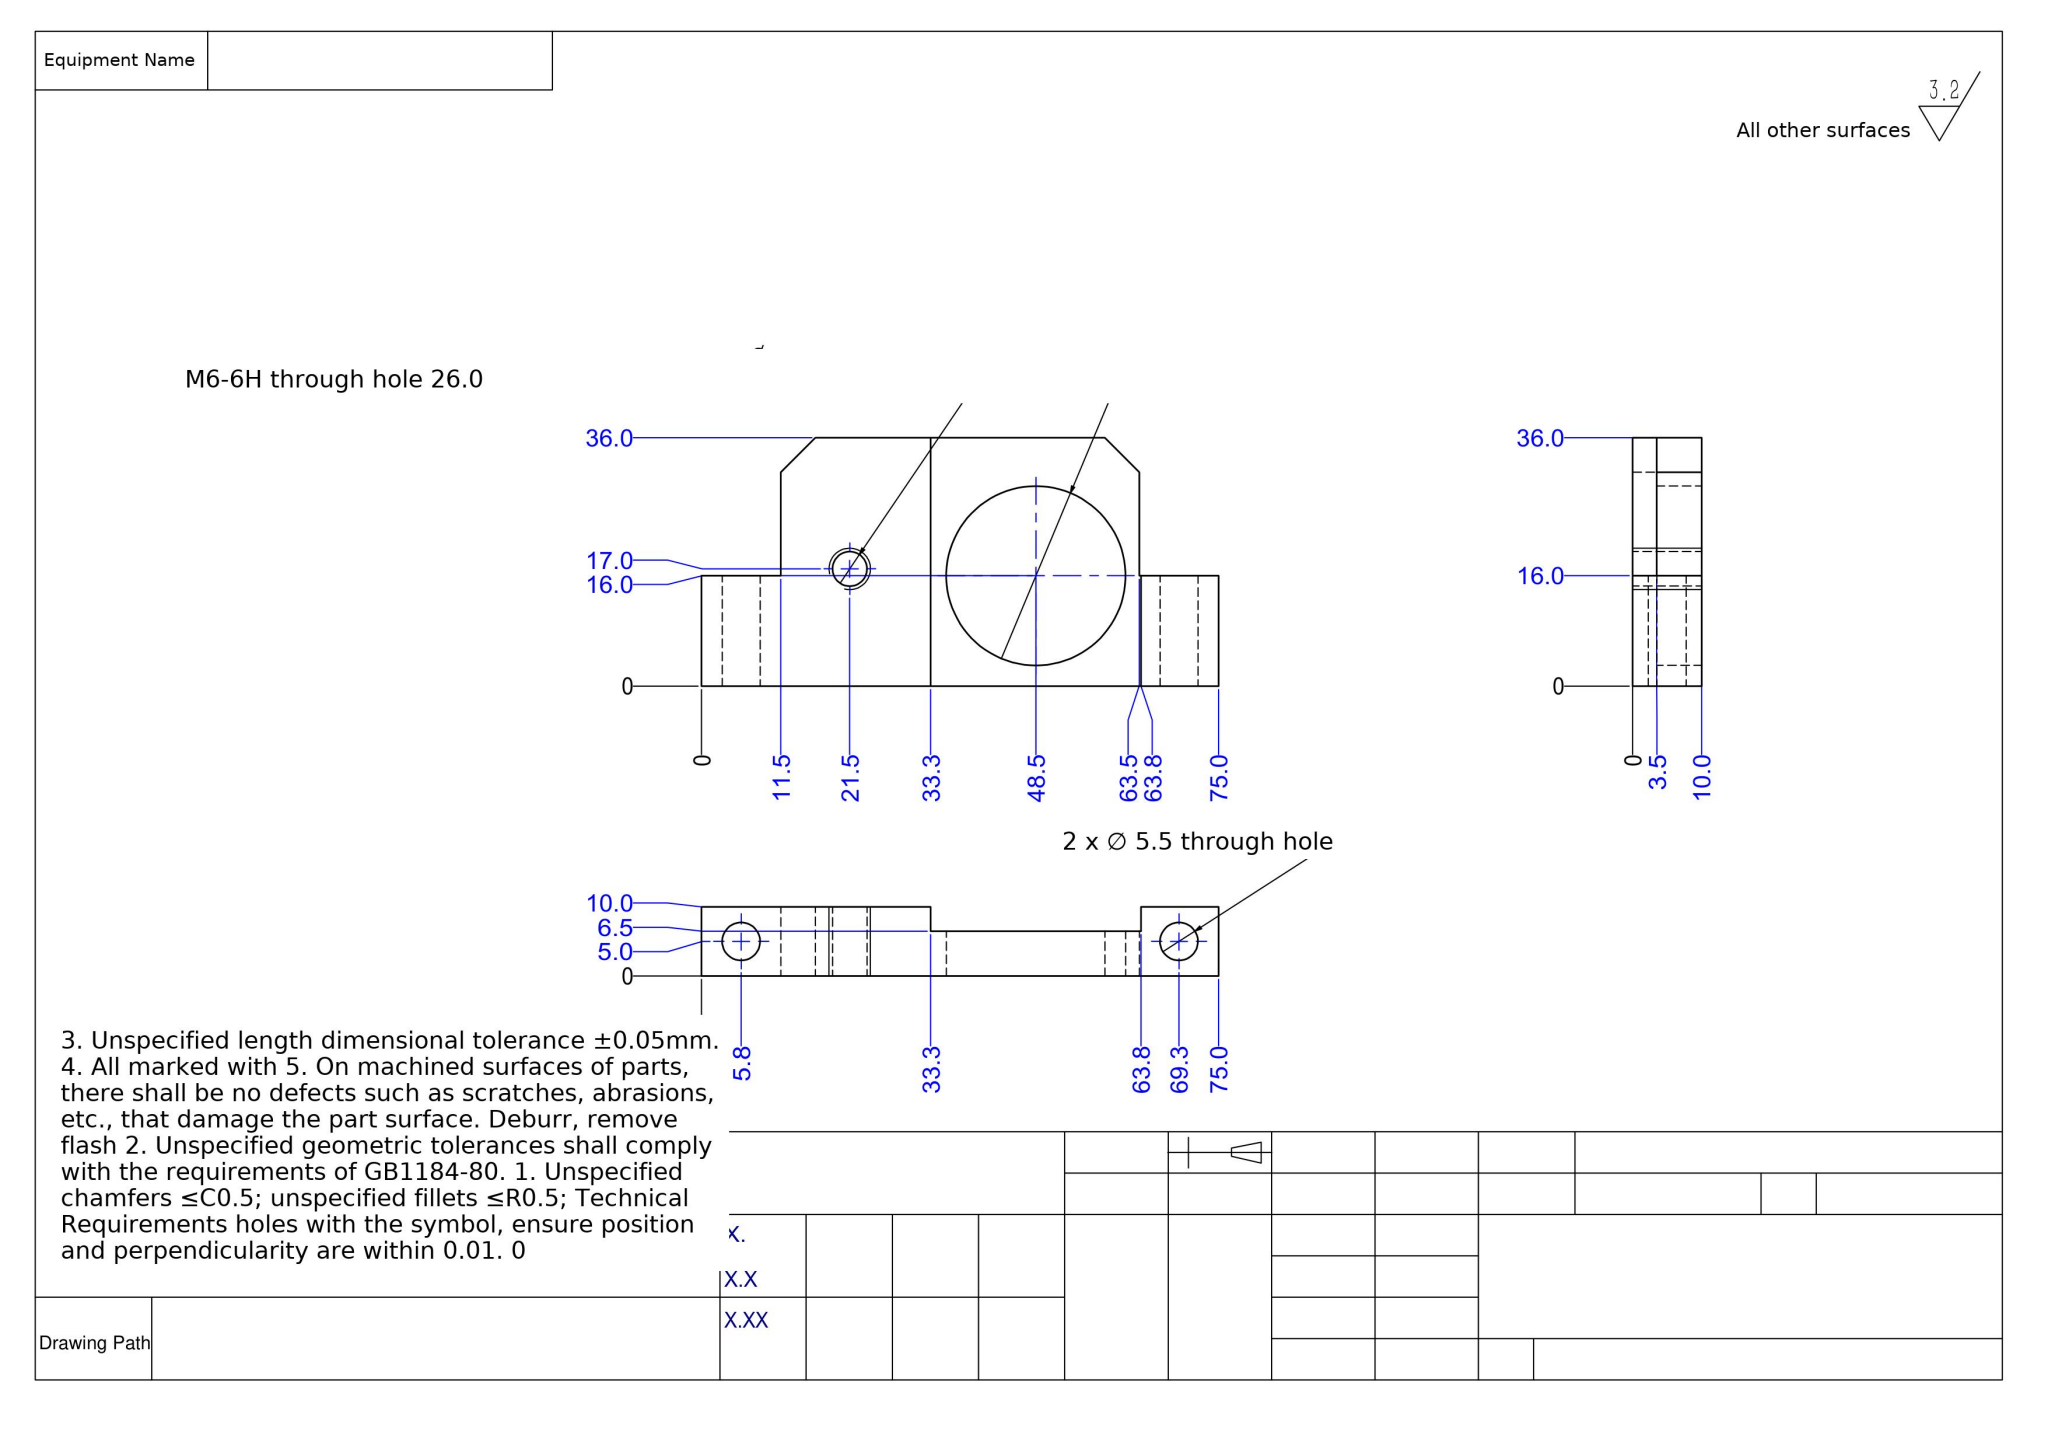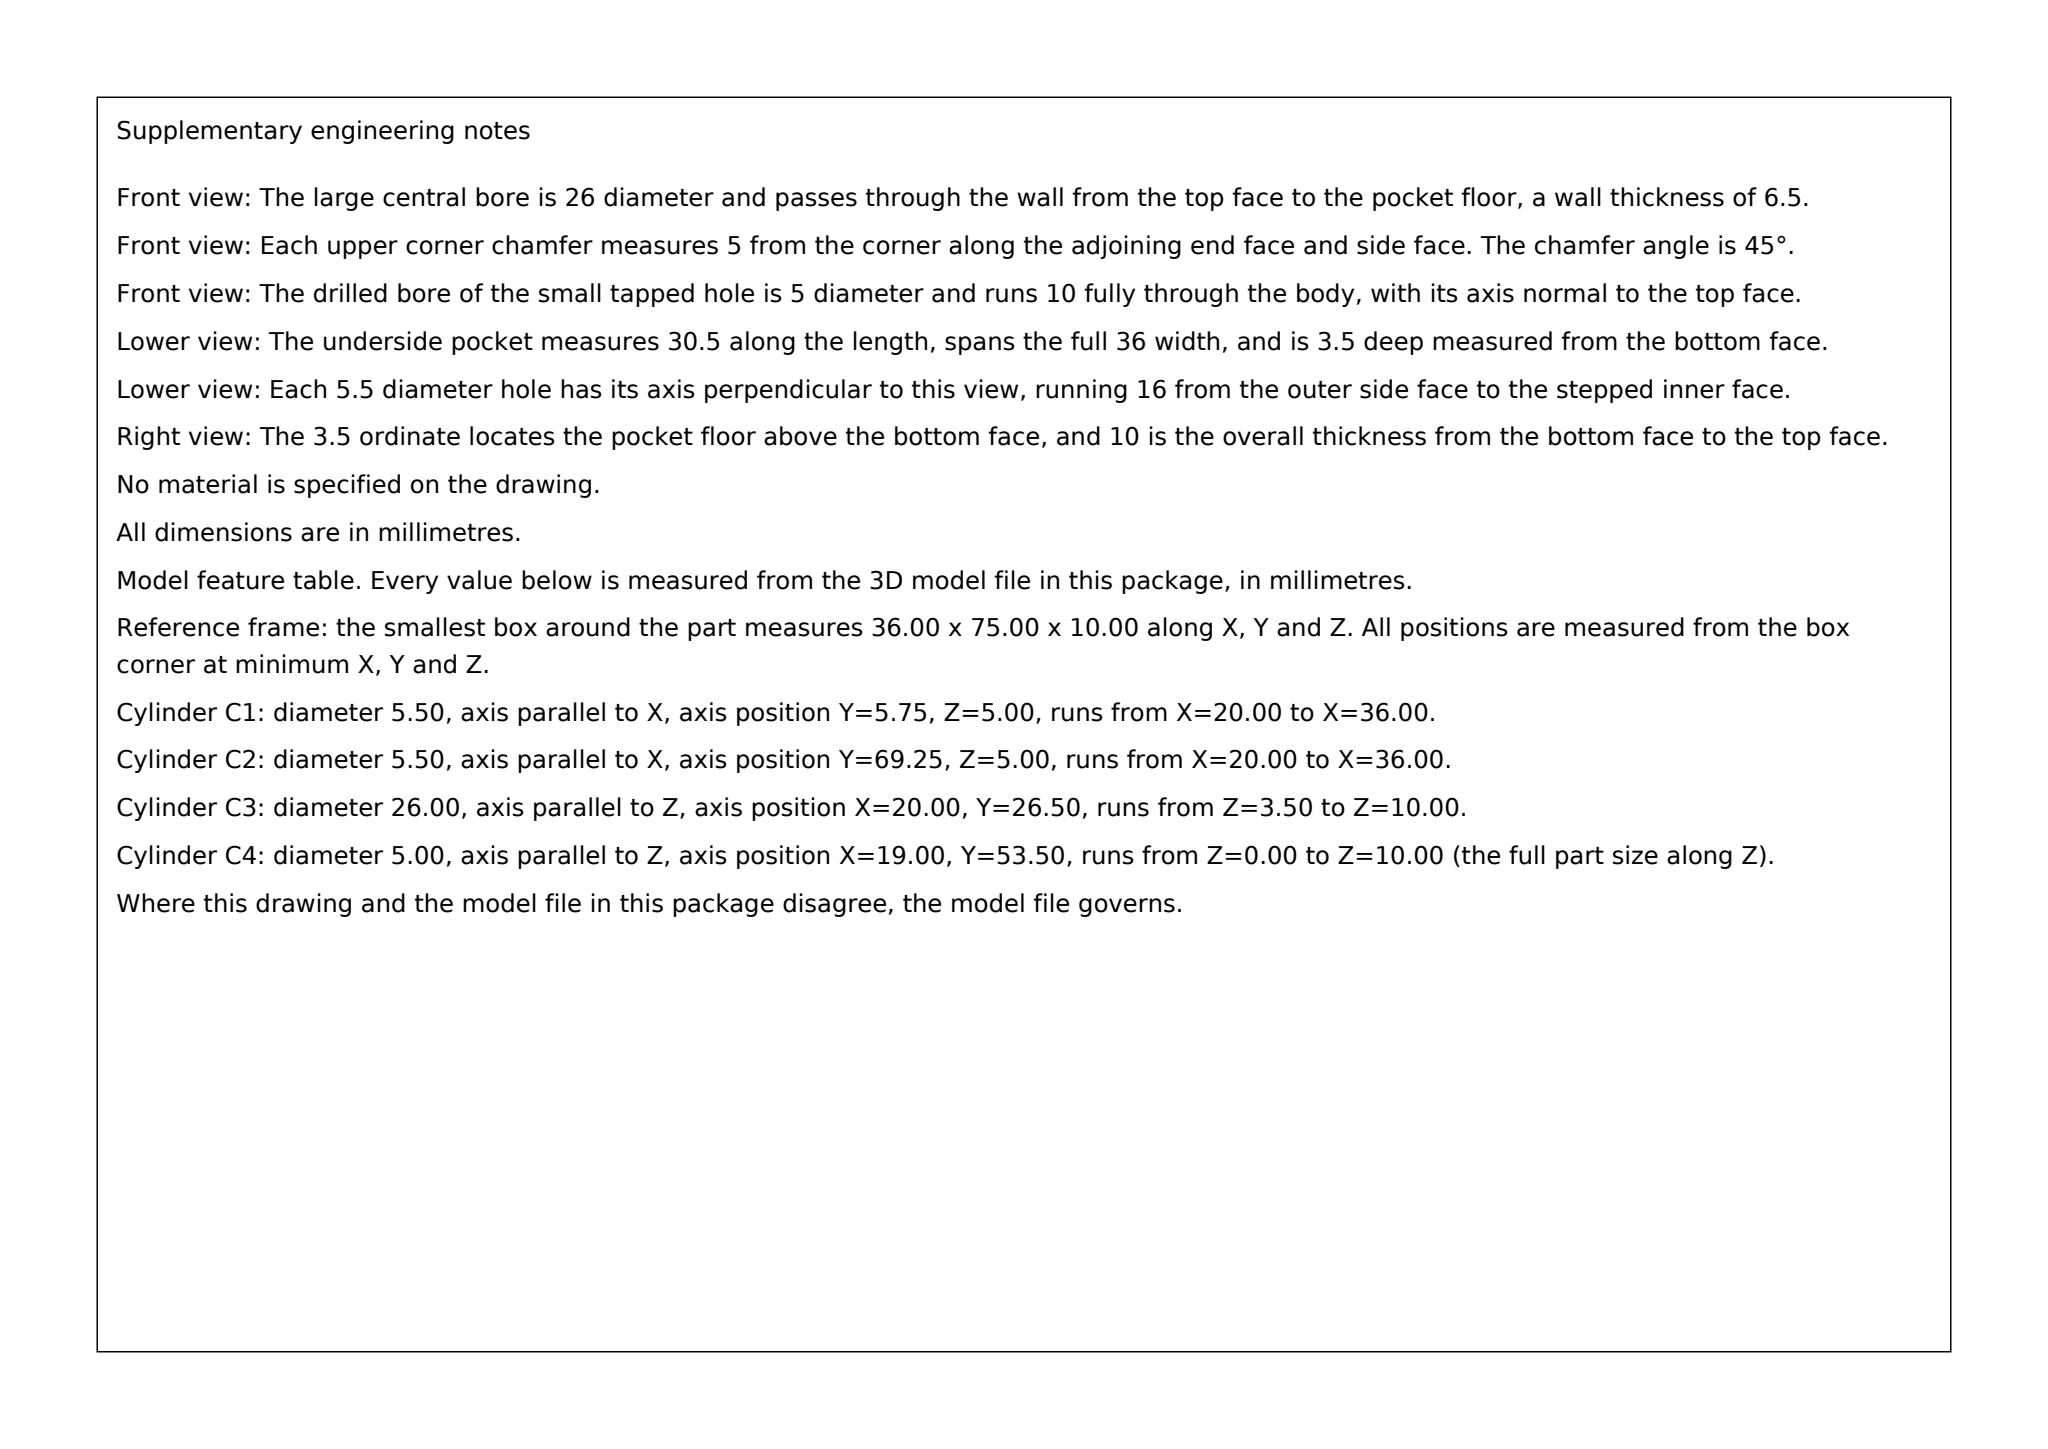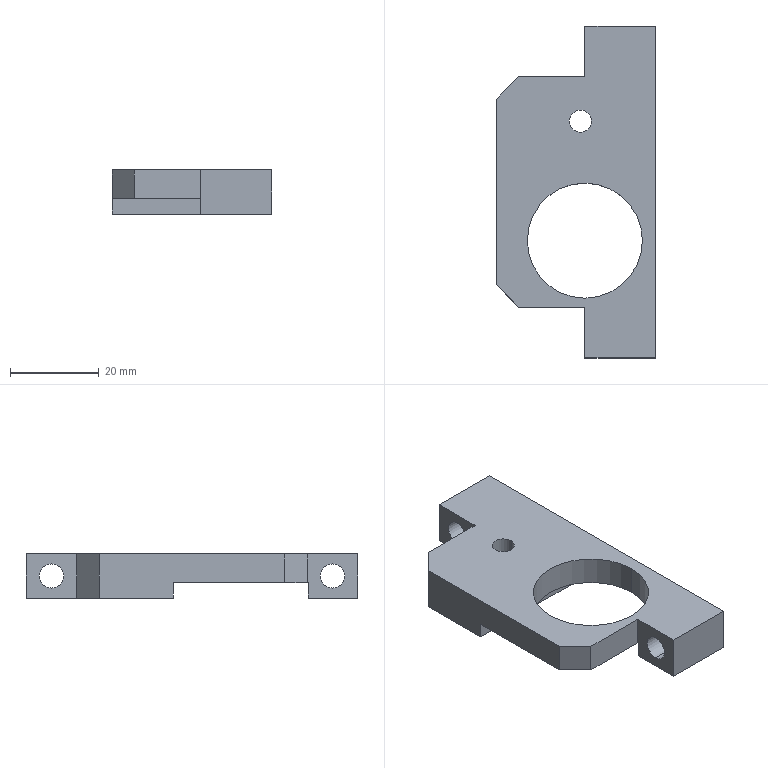Part | SolidWorks | mm | 1 solid | 24 faces | box 36 x 75 x 10 mm | volume 13961 mm3 | plane 16 | cylinder 8 | commonest cylinder face diameters 5.5 x4 5 x2 26 x2
Drawing notes:
FRONT VIEW: 2 X C5 ON TOP CORNERS OF 36.0 FACE (AT 11.5 & 63.5) | from the solid: Top face (x=0 plane, drawing 36.0) spans y 16.5-58.5 between the 11.5 and 63.5 side faces (step y=63.5 / 11.5), i.e. 5 mm x 45 deg cut at each top corner of the 52 wide block.
Ø26 BORE DP 6.5 FROM TOP FACE, CL AT 48.5; FLOOR AT 3.5 | from the solid: cyl dia 26, axis z, pos (20,26.5), len 6.5; z planes 3.5 & 10.0; 75-26.5=48.5
Ø5.0 THRU, CL AT 21.5 & 17.0 (FRONT VIEW) | from the solid: cyl dia 5.0, axis z, pos (19,53.5), len 10.0 = full 10 thk; 75-53.5=21.5, 36-19=17.0
TECH REQ: MARKED HOLES POS & PERP W/IN 0.01; LEN TOL ±0.05 | from the solid: note block text; Ø5.0 THRU holes full 10 thk through part, bbox 36x75x10
build123d program:
from build123d import *

# Parameters (mm, degrees)
SKETCH1_W            = 36
SKETCH1_H            = 75
BOSS_EXTRUDE1_DEPTH  = 10
SKETCH2_W            = 20
SKETCH2_H            = 11.5
CUT_EXTRUDE1_DEPTH   = 43.781
SKETCH3_R            = 13
CUT_EXTRUDE2_DEPTH   = 43.781
M6_TAPPED_HOLE1_D    = 5
CHAMFER1_SIZE        = 5
M5_CLEARANCE_HOLE1_D = 5.5
SKETCH8_W            = 40
SKETCH8_H            = 30.5
CUT_EXTRUDE3_DEPTH   = 3.5


with BuildPart() as part:
    # Sketch1 → Boss-Extrude1 (new body)
    with BuildSketch(Plane.XY):
        Rectangle(SKETCH1_W, SKETCH1_H)
    extrude(amount=BOSS_EXTRUDE1_DEPTH)

    # Sketch2 → Cut-Extrude1 (cut, through all)
    with BuildSketch(Plane.XY.offset(10)):
        with Locations((-8, 31.75)):
            Rectangle(SKETCH2_W, SKETCH2_H)
        with Locations((-8, -31.75)):
            Rectangle(SKETCH2_W, SKETCH2_H)
    extrude(amount=-CUT_EXTRUDE1_DEPTH, mode=Mode.SUBTRACT)

    # Sketch3 → Cut-Extrude2 (cut, through all)
    with BuildSketch(Plane.XY.offset(10)):
        with Locations((2, -11)):
            Circle(SKETCH3_R)
    extrude(amount=-CUT_EXTRUDE2_DEPTH, mode=Mode.SUBTRACT)

    # M6 Tapped Hole1 (through all)
    with Locations(Plane.XY.offset(10)):
        with Locations((1, 16)):
            Hole(M6_TAPPED_HOLE1_D / 2)

    # Chamfer1
    chamfer1_edges = [part.edges().sort_by_distance(p)[0] for p in [
        (-18, 26, 5),
        (-18, -26, 5),
    ]]
    chamfer(chamfer1_edges, length=CHAMFER1_SIZE)

    # M5 Clearance Hole1 (through all)
    with Locations(Plane.ZY.offset(-2)):
        with Locations((5, -31.75), (5, 31.75)):
            Hole(M5_CLEARANCE_HOLE1_D / 2)

    # Sketch8 → Cut-Extrude3 (cut)
    with BuildSketch(Plane(origin=(0, 0, 0), x_dir=(-1, 0, 0), z_dir=(0, 0, -1))):
        with Locations((-2, -11)):
            Rectangle(SKETCH8_W, SKETCH8_H)
    extrude(amount=-CUT_EXTRUDE3_DEPTH, mode=Mode.SUBTRACT)


solid = part.part
STEP:
#1=CARTESIAN_POINT('',(18.,-31.75,2.25));
#2=VERTEX_POINT('',#1);
#3=CARTESIAN_POINT('',(18.,-31.75,7.75));
#4=VERTEX_POINT('',#3);
#5=CARTESIAN_POINT('',(18.,-31.75,5.));
#6=DIRECTION('',(-1.,0.,0.));
#7=DIRECTION('',(0.,0.,1.));
#8=AXIS2_PLACEMENT_3D('',#5,#6,#7);
#9=CIRCLE('',#8,2.75);
#10=EDGE_CURVE('',#2,#4,#9,.T.);
#11=ORIENTED_EDGE('',*,*,#10,.F.);
#12=CARTESIAN_POINT('',(2.,-31.75,2.25));
#13=VERTEX_POINT('',#12);
#14=CARTESIAN_POINT('',(2.,-31.75,2.25));
#15=DIRECTION('',(-1.,0.,0.));
#16=VECTOR('',#15,1000.);
#17=LINE('',#14,#16);
#18=EDGE_CURVE('',#2,#13,#17,.T.);
#19=ORIENTED_EDGE('',*,*,#18,.T.);
#20=CARTESIAN_POINT('',(2.,-31.75,7.75));
#21=VERTEX_POINT('',#20);
#22=CARTESIAN_POINT('',(2.,-31.75,5.));
#23=DIRECTION('',(-1.,0.,0.));
#24=DIRECTION('',(0.,0.,1.));
#25=AXIS2_PLACEMENT_3D('',#22,#23,#24);
#26=CIRCLE('',#25,2.75);
#27=EDGE_CURVE('',#13,#21,#26,.T.);
#28=ORIENTED_EDGE('',*,*,#27,.T.);
#29=CARTESIAN_POINT('',(2.,-31.75,7.75));
#30=DIRECTION('',(-1.,0.,0.));
#31=VECTOR('',#30,1000.);
#32=LINE('',#29,#31);
#33=EDGE_CURVE('',#4,#21,#32,.T.);
#34=ORIENTED_EDGE('',*,*,#33,.F.);
#35=EDGE_LOOP('',(#11,#19,#28,#34));
#36=FACE_OUTER_BOUND('',#35,.T.);
#37=CARTESIAN_POINT('',(2.,-31.75,5.));
#38=DIRECTION('',(-1.,0.,0.));
#39=DIRECTION('',(0.,0.,1.));
#40=AXIS2_PLACEMENT_3D('',#37,#38,#39);
#41=CYLINDRICAL_SURFACE('',#40,2.75);
#42=ADVANCED_FACE('',(#36),#41,.F.);
#43=CARTESIAN_POINT('',(18.,31.75,2.25));
#44=VERTEX_POINT('',#43);
#45=CARTESIAN_POINT('',(18.,31.75,7.75));
#46=VERTEX_POINT('',#45);
#47=CARTESIAN_POINT('',(18.,31.75,5.));
#48=DIRECTION('',(-1.,0.,0.));
#49=DIRECTION('',(0.,0.,1.));
#50=AXIS2_PLACEMENT_3D('',#47,#48,#49);
#51=CIRCLE('',#50,2.75);
#52=EDGE_CURVE('',#44,#46,#51,.T.);
#53=ORIENTED_EDGE('',*,*,#52,.F.);
#54=CARTESIAN_POINT('',(2.,31.75,2.25));
#55=VERTEX_POINT('',#54);
#56=CARTESIAN_POINT('',(2.,31.75,2.25));
#57=DIRECTION('',(-1.,0.,0.));
#58=VECTOR('',#57,1000.);
#59=LINE('',#56,#58);
#60=EDGE_CURVE('',#44,#55,#59,.T.);
#61=ORIENTED_EDGE('',*,*,#60,.T.);
#62=CARTESIAN_POINT('',(2.,31.75,7.75));
#63=VERTEX_POINT('',#62);
#64=CARTESIAN_POINT('',(2.,31.75,5.));
#65=DIRECTION('',(-1.,0.,0.));
#66=DIRECTION('',(0.,0.,1.));
#67=AXIS2_PLACEMENT_3D('',#64,#65,#66);
#68=CIRCLE('',#67,2.75);
#69=EDGE_CURVE('',#55,#63,#68,.T.);
#70=ORIENTED_EDGE('',*,*,#69,.T.);
#71=CARTESIAN_POINT('',(2.,31.75,7.75));
#72=DIRECTION('',(-1.,0.,0.));
#73=VECTOR('',#72,1000.);
#74=LINE('',#71,#73);
#75=EDGE_CURVE('',#46,#63,#74,.T.);
#76=ORIENTED_EDGE('',*,*,#75,.F.);
#77=EDGE_LOOP('',(#53,#61,#70,#76));
#78=FACE_OUTER_BOUND('',#77,.T.);
#79=CARTESIAN_POINT('',(2.,31.75,5.));
#80=DIRECTION('',(-1.,0.,0.));
#81=DIRECTION('',(0.,0.,1.));
#82=AXIS2_PLACEMENT_3D('',#79,#80,#81);
#83=CYLINDRICAL_SURFACE('',#82,2.75);
#84=ADVANCED_FACE('',(#78),#83,.F.);
#85=CARTESIAN_POINT('',(-1.5,16.,0.));
#86=VERTEX_POINT('',#85);
#87=CARTESIAN_POINT('',(3.5,16.,0.));
#88=VERTEX_POINT('',#87);
#89=CARTESIAN_POINT('',(1.,16.,0.));
#90=DIRECTION('',(0.,0.,1.));
#91=DIRECTION('',(1.,0.,0.));
#92=AXIS2_PLACEMENT_3D('',#89,#90,#91);
#93=CIRCLE('',#92,2.5);
#94=EDGE_CURVE('',#86,#88,#93,.T.);
#95=ORIENTED_EDGE('',*,*,#94,.F.);
#96=CARTESIAN_POINT('',(-1.5,16.,10.));
#97=VERTEX_POINT('',#96);
#98=CARTESIAN_POINT('',(-1.5,16.,10.));
#99=DIRECTION('',(0.,0.,1.));
#100=VECTOR('',#99,1000.);
#101=LINE('',#98,#100);
#102=EDGE_CURVE('',#86,#97,#101,.T.);
#103=ORIENTED_EDGE('',*,*,#102,.T.);
#104=CARTESIAN_POINT('',(3.5,16.,10.));
#105=VERTEX_POINT('',#104);
#106=CARTESIAN_POINT('',(1.,16.,10.));
#107=DIRECTION('',(0.,0.,1.));
#108=DIRECTION('',(1.,0.,0.));
#109=AXIS2_PLACEMENT_3D('',#106,#107,#108);
#110=CIRCLE('',#109,2.5);
#111=EDGE_CURVE('',#97,#105,#110,.T.);
#112=ORIENTED_EDGE('',*,*,#111,.T.);
#113=CARTESIAN_POINT('',(3.5,16.,10.));
#114=DIRECTION('',(0.,0.,1.));
#115=VECTOR('',#114,1000.);
#116=LINE('',#113,#115);
#117=EDGE_CURVE('',#88,#105,#116,.T.);
#118=ORIENTED_EDGE('',*,*,#117,.F.);
#119=EDGE_LOOP('',(#95,#103,#112,#118));
#120=FACE_OUTER_BOUND('',#119,.T.);
#121=CARTESIAN_POINT('',(1.,16.,10.));
#122=DIRECTION('',(0.,0.,1.));
#123=DIRECTION('',(1.,0.,0.));
#124=AXIS2_PLACEMENT_3D('',#121,#122,#123);
#125=CYLINDRICAL_SURFACE('',#124,2.5);
#126=ADVANCED_FACE('',(#120),#125,.F.);
#127=CARTESIAN_POINT('',(-11.,-11.,3.5));
#128=VERTEX_POINT('',#127);
#129=CARTESIAN_POINT('',(15.,-11.,3.5));
#130=VERTEX_POINT('',#129);
#131=CARTESIAN_POINT('',(2.,-11.,3.5));
#132=DIRECTION('',(0.,0.,1.));
#133=DIRECTION('',(-1.,0.,0.));
#134=AXIS2_PLACEMENT_3D('',#131,#132,#133);
#135=CIRCLE('',#134,13.);
#136=EDGE_CURVE('',#128,#130,#135,.T.);
#137=ORIENTED_EDGE('',*,*,#136,.F.);
#138=CARTESIAN_POINT('',(-11.,-11.,10.));
#139=VERTEX_POINT('',#138);
#140=CARTESIAN_POINT('',(-11.,-11.,0.));
#141=DIRECTION('',(0.,0.,1.));
#142=VECTOR('',#141,1000.);
#143=LINE('',#140,#142);
#144=EDGE_CURVE('',#128,#139,#143,.T.);
#145=ORIENTED_EDGE('',*,*,#144,.T.);
#146=CARTESIAN_POINT('',(15.,-11.,10.));
#147=VERTEX_POINT('',#146);
#148=CARTESIAN_POINT('',(2.,-11.,10.));
#149=DIRECTION('',(0.,0.,1.));
#150=DIRECTION('',(1.,0.,0.));
#151=AXIS2_PLACEMENT_3D('',#148,#149,#150);
#152=CIRCLE('',#151,13.);
#153=EDGE_CURVE('',#139,#147,#152,.T.);
#154=ORIENTED_EDGE('',*,*,#153,.T.);
#155=CARTESIAN_POINT('',(15.,-11.,0.));
#156=DIRECTION('',(0.,0.,1.));
#157=VECTOR('',#156,1000.);
#158=LINE('',#155,#157);
#159=EDGE_CURVE('',#130,#147,#158,.T.);
#160=ORIENTED_EDGE('',*,*,#159,.F.);
#161=EDGE_LOOP('',(#137,#145,#154,#160));
#162=FACE_OUTER_BOUND('',#161,.T.);
#163=CARTESIAN_POINT('',(2.,-11.,0.));
#164=DIRECTION('',(0.,0.,1.));
#165=DIRECTION('',(1.,0.,0.));
#166=AXIS2_PLACEMENT_3D('',#163,#164,#165);
#167=CYLINDRICAL_SURFACE('',#166,13.);
#168=ADVANCED_FACE('',(#162),#167,.F.);
#169=CARTESIAN_POINT('',(2.,-37.5,0.));
#170=VERTEX_POINT('',#169);
#171=CARTESIAN_POINT('',(2.,-26.25,0.));
#172=VERTEX_POINT('',#171);
#173=CARTESIAN_POINT('',(2.,-37.5,0.));
#174=DIRECTION('',(0.,1.,0.));
#175=VECTOR('',#174,1000.);
#176=LINE('',#173,#175);
#177=EDGE_CURVE('',#170,#172,#176,.T.);
#178=ORIENTED_EDGE('',*,*,#177,.T.);
#179=CARTESIAN_POINT('',(18.,-26.25,0.));
#180=VERTEX_POINT('',#179);
#181=CARTESIAN_POINT('',(22.,-26.25,0.));
#182=DIRECTION('',(-1.,0.,0.));
#183=VECTOR('',#182,1000.);
#184=LINE('',#181,#183);
#185=EDGE_CURVE('',#180,#172,#184,.T.);
#186=ORIENTED_EDGE('',*,*,#185,.F.);
#187=CARTESIAN_POINT('',(18.,-37.5,0.));
#188=VERTEX_POINT('',#187);
#189=CARTESIAN_POINT('',(18.,37.5,0.));
#190=DIRECTION('',(-0.,1.,0.));
#191=VECTOR('',#190,1000.);
#192=LINE('',#189,#191);
#193=EDGE_CURVE('',#188,#180,#192,.T.);
#194=ORIENTED_EDGE('',*,*,#193,.F.);
#195=CARTESIAN_POINT('',(-18.,-37.5,0.));
#196=DIRECTION('',(1.,0.,0.));
#197=VECTOR('',#196,1000.);
#198=LINE('',#195,#197);
#199=EDGE_CURVE('',#170,#188,#198,.T.);
#200=ORIENTED_EDGE('',*,*,#199,.F.);
#201=EDGE_LOOP('',(#178,#186,#194,#200));
#202=FACE_OUTER_BOUND('',#201,.T.);
#203=CARTESIAN_POINT('',(0.,0.,0.));
#204=DIRECTION('',(0.,0.,1.));
#205=DIRECTION('',(1.,0.,0.));
#206=AXIS2_PLACEMENT_3D('',#203,#204,#205);
#207=PLANE('',#206);
#208=ADVANCED_FACE('',(#202),#207,.F.);
#209=CARTESIAN_POINT('',(2.,-26.,3.5));
#210=VERTEX_POINT('',#209);
#211=CARTESIAN_POINT('',(-13.,-26.,3.5));
#212=VERTEX_POINT('',#211);
#213=CARTESIAN_POINT('',(-18.,-26.,3.5));
#214=DIRECTION('',(-1.,-0.,0.));
#215=VECTOR('',#214,1000.);
#216=LINE('',#213,#215);
#217=EDGE_CURVE('',#210,#212,#216,.T.);
#218=ORIENTED_EDGE('',*,*,#217,.F.);
#219=CARTESIAN_POINT('',(2.,-26.,10.));
#220=VERTEX_POINT('',#219);
#221=CARTESIAN_POINT('',(2.,-26.,0.));
#222=DIRECTION('',(0.,0.,1.));
#223=VECTOR('',#222,1000.);
#224=LINE('',#221,#223);
#225=EDGE_CURVE('',#210,#220,#224,.T.);
#226=ORIENTED_EDGE('',*,*,#225,.T.);
#227=CARTESIAN_POINT('',(-13.,-26.,10.));
#228=VERTEX_POINT('',#227);
#229=CARTESIAN_POINT('',(-18.,-26.,10.));
#230=DIRECTION('',(-1.,-0.,0.));
#231=VECTOR('',#230,1000.);
#232=LINE('',#229,#231);
#233=EDGE_CURVE('',#220,#228,#232,.T.);
#234=ORIENTED_EDGE('',*,*,#233,.T.);
#235=CARTESIAN_POINT('',(-13.,-26.,0.));
#236=DIRECTION('',(0.,0.,-1.));
#237=VECTOR('',#236,1000.);
#238=LINE('',#235,#237);
#239=EDGE_CURVE('',#228,#212,#238,.T.);
#240=ORIENTED_EDGE('',*,*,#239,.T.);
#241=EDGE_LOOP('',(#218,#226,#234,#240));
#242=FACE_OUTER_BOUND('',#241,.T.);
#243=CARTESIAN_POINT('',(-18.,-26.,0.));
#244=DIRECTION('',(-0.,1.,0.));
#245=DIRECTION('',(-1.,-0.,0.));
#246=AXIS2_PLACEMENT_3D('',#243,#244,#245);
#247=PLANE('',#246);
#248=ADVANCED_FACE('',(#242),#247,.F.);
#249=ORIENTED_EDGE('',*,*,#144,.F.);
#250=CARTESIAN_POINT('',(2.,-11.,3.5));
#251=DIRECTION('',(0.,0.,1.));
#252=DIRECTION('',(-1.,0.,0.));
#253=AXIS2_PLACEMENT_3D('',#250,#251,#252);
#254=CIRCLE('',#253,13.);
#255=EDGE_CURVE('',#130,#128,#254,.T.);
#256=ORIENTED_EDGE('',*,*,#255,.F.);
#257=ORIENTED_EDGE('',*,*,#159,.T.);
#258=CARTESIAN_POINT('',(2.,-11.,10.));
#259=DIRECTION('',(0.,0.,1.));
#260=DIRECTION('',(1.,0.,0.));
#261=AXIS2_PLACEMENT_3D('',#258,#259,#260);
#262=CIRCLE('',#261,13.);
#263=EDGE_CURVE('',#147,#139,#262,.T.);
#264=ORIENTED_EDGE('',*,*,#263,.T.);
#265=EDGE_LOOP('',(#249,#256,#257,#264));
#266=FACE_OUTER_BOUND('',#265,.T.);
#267=CARTESIAN_POINT('',(2.,-11.,0.));
#268=DIRECTION('',(0.,0.,1.));
#269=DIRECTION('',(1.,0.,0.));
#270=AXIS2_PLACEMENT_3D('',#267,#268,#269);
#271=CYLINDRICAL_SURFACE('',#270,13.);
#272=ADVANCED_FACE('',(#266),#271,.F.);
#273=CARTESIAN_POINT('',(-18.,-21.,3.5));
#274=VERTEX_POINT('',#273);
#275=CARTESIAN_POINT('',(-18.,-21.,10.));
#276=VERTEX_POINT('',#275);
#277=CARTESIAN_POINT('',(-18.,-21.,10.));
#278=DIRECTION('',(0.,0.,1.));
#279=VECTOR('',#278,1000.);
#280=LINE('',#277,#279);
#281=EDGE_CURVE('',#274,#276,#280,.T.);
#282=ORIENTED_EDGE('',*,*,#281,.F.);
#283=CARTESIAN_POINT('',(-18.,-21.,3.5));
#284=DIRECTION('',(0.7071,-0.7071,0.));
#285=VECTOR('',#284,1000.);
#286=LINE('',#283,#285);
#287=EDGE_CURVE('',#274,#212,#286,.T.);
#288=ORIENTED_EDGE('',*,*,#287,.T.);
#289=ORIENTED_EDGE('',*,*,#239,.F.);
#290=CARTESIAN_POINT('',(-19.5,-19.5,10.));
#291=DIRECTION('',(0.7071,-0.7071,0.));
#292=VECTOR('',#291,1000.);
#293=LINE('',#290,#292);
#294=EDGE_CURVE('',#276,#228,#293,.T.);
#295=ORIENTED_EDGE('',*,*,#294,.F.);
#296=EDGE_LOOP('',(#282,#288,#289,#295));
#297=FACE_OUTER_BOUND('',#296,.T.);
#298=CARTESIAN_POINT('',(-18.,-21.,10.));
#299=DIRECTION('',(0.7071,0.7071,0.));
#300=DIRECTION('',(0.,0.,1.));
#301=AXIS2_PLACEMENT_3D('',#298,#299,#300);
#302=PLANE('',#301);
#303=ADVANCED_FACE('',(#297),#302,.F.);
#304=ORIENTED_EDGE('',*,*,#193,.T.);
#305=CARTESIAN_POINT('',(18.,-26.25,3.5));
#306=VERTEX_POINT('',#305);
#307=CARTESIAN_POINT('',(18.,-26.25,10.));
#308=DIRECTION('',(0.,0.,1.));
#309=VECTOR('',#308,1000.);
#310=LINE('',#307,#309);
#311=EDGE_CURVE('',#180,#306,#310,.T.);
#312=ORIENTED_EDGE('',*,*,#311,.T.);
#313=CARTESIAN_POINT('',(18.,4.25,3.5));
#314=VERTEX_POINT('',#313);
#315=CARTESIAN_POINT('',(18.,37.5,3.5));
#316=DIRECTION('',(0.,-1.,0.));
#317=VECTOR('',#316,1000.);
#318=LINE('',#315,#317);
#319=EDGE_CURVE('',#314,#306,#318,.T.);
#320=ORIENTED_EDGE('',*,*,#319,.F.);
#321=CARTESIAN_POINT('',(18.,4.25,0.));
#322=VERTEX_POINT('',#321);
#323=CARTESIAN_POINT('',(18.,4.25,10.));
#324=DIRECTION('',(0.,0.,-1.));
#325=VECTOR('',#324,1000.);
#326=LINE('',#323,#325);
#327=EDGE_CURVE('',#314,#322,#326,.T.);
#328=ORIENTED_EDGE('',*,*,#327,.T.);
#329=CARTESIAN_POINT('',(18.,37.5,0.));
#330=VERTEX_POINT('',#329);
#331=CARTESIAN_POINT('',(18.,37.5,0.));
#332=DIRECTION('',(-0.,1.,0.));
#333=VECTOR('',#332,1000.);
#334=LINE('',#331,#333);
#335=EDGE_CURVE('',#322,#330,#334,.T.);
#336=ORIENTED_EDGE('',*,*,#335,.T.);
#337=CARTESIAN_POINT('',(18.,37.5,10.));
#338=VERTEX_POINT('',#337);
#339=CARTESIAN_POINT('',(18.,37.5,10.));
#340=DIRECTION('',(0.,0.,-1.));
#341=VECTOR('',#340,1000.);
#342=LINE('',#339,#341);
#343=EDGE_CURVE('',#338,#330,#342,.T.);
#344=ORIENTED_EDGE('',*,*,#343,.F.);
#345=CARTESIAN_POINT('',(18.,-37.5,10.));
#346=VERTEX_POINT('',#345);
#347=CARTESIAN_POINT('',(18.,37.5,10.));
#348=DIRECTION('',(-0.,1.,0.));
#349=VECTOR('',#348,1000.);
#350=LINE('',#347,#349);
#351=EDGE_CURVE('',#346,#338,#350,.T.);
#352=ORIENTED_EDGE('',*,*,#351,.F.);
#353=CARTESIAN_POINT('',(18.,-37.5,10.));
#354=DIRECTION('',(0.,0.,-1.));
#355=VECTOR('',#354,1000.);
#356=LINE('',#353,#355);
#357=EDGE_CURVE('',#346,#188,#356,.T.);
#358=ORIENTED_EDGE('',*,*,#357,.T.);
#359=EDGE_LOOP('',(#304,#312,#320,#328,#336,#344,#352,#358));
#360=FACE_OUTER_BOUND('',#359,.T.);
#361=CARTESIAN_POINT('',(18.,-31.75,5.));
#362=DIRECTION('',(-1.,0.,0.));
#363=DIRECTION('',(0.,0.,1.));
#364=AXIS2_PLACEMENT_3D('',#361,#362,#363);
#365=CIRCLE('',#364,2.75);
#366=EDGE_CURVE('',#4,#2,#365,.T.);
#367=ORIENTED_EDGE('',*,*,#366,.T.);
#368=ORIENTED_EDGE('',*,*,#10,.T.);
#369=EDGE_LOOP('',(#367,#368));
#370=FACE_BOUND('',#369,.T.);
#371=CARTESIAN_POINT('',(18.,31.75,5.));
#372=DIRECTION('',(-1.,0.,0.));
#373=DIRECTION('',(0.,0.,1.));
#374=AXIS2_PLACEMENT_3D('',#371,#372,#373);
#375=CIRCLE('',#374,2.75);
#376=EDGE_CURVE('',#46,#44,#375,.T.);
#377=ORIENTED_EDGE('',*,*,#376,.T.);
#378=ORIENTED_EDGE('',*,*,#52,.T.);
#379=EDGE_LOOP('',(#377,#378));
#380=FACE_BOUND('',#379,.T.);
#381=CARTESIAN_POINT('',(18.,37.5,10.));
#382=DIRECTION('',(-1.,-0.,0.));
#383=DIRECTION('',(0.,-1.,0.));
#384=AXIS2_PLACEMENT_3D('',#381,#382,#383);
#385=PLANE('',#384);
#386=ADVANCED_FACE('',(#360,#370,#380),#385,.F.);
#387=CARTESIAN_POINT('',(2.,37.5,0.));
#388=VERTEX_POINT('',#387);
#389=CARTESIAN_POINT('',(-18.,37.5,0.));
#390=DIRECTION('',(-1.,0.,0.));
#391=VECTOR('',#390,1000.);
#392=LINE('',#389,#391);
#393=EDGE_CURVE('',#330,#388,#392,.T.);
#394=ORIENTED_EDGE('',*,*,#393,.T.);
#395=CARTESIAN_POINT('',(2.,37.5,10.));
#396=VERTEX_POINT('',#395);
#397=CARTESIAN_POINT('',(2.,37.5,0.));
#398=DIRECTION('',(0.,0.,1.));
#399=VECTOR('',#398,1000.);
#400=LINE('',#397,#399);
#401=EDGE_CURVE('',#388,#396,#400,.T.);
#402=ORIENTED_EDGE('',*,*,#401,.T.);
#403=CARTESIAN_POINT('',(-18.,37.5,10.));
#404=DIRECTION('',(-1.,0.,0.));
#405=VECTOR('',#404,1000.);
#406=LINE('',#403,#405);
#407=EDGE_CURVE('',#338,#396,#406,.T.);
#408=ORIENTED_EDGE('',*,*,#407,.F.);
#409=ORIENTED_EDGE('',*,*,#343,.T.);
#410=EDGE_LOOP('',(#394,#402,#408,#409));
#411=FACE_OUTER_BOUND('',#410,.T.);
#412=CARTESIAN_POINT('',(-18.,37.5,10.));
#413=DIRECTION('',(0.,-1.,0.));
#414=DIRECTION('',(0.,0.,-1.));
#415=AXIS2_PLACEMENT_3D('',#412,#413,#414);
#416=PLANE('',#415);
#417=ADVANCED_FACE('',(#411),#416,.F.);
#418=CARTESIAN_POINT('',(-18.,21.,0.));
#419=VERTEX_POINT('',#418);
#420=CARTESIAN_POINT('',(-18.,4.25,0.));
#421=VERTEX_POINT('',#420);
#422=CARTESIAN_POINT('',(-18.,37.5,0.));
#423=DIRECTION('',(0.,-1.,0.));
#424=VECTOR('',#423,1000.);
#425=LINE('',#422,#424);
#426=EDGE_CURVE('',#419,#421,#425,.T.);
#427=ORIENTED_EDGE('',*,*,#426,.T.);
#428=CARTESIAN_POINT('',(-18.,4.25,3.5));
#429=VERTEX_POINT('',#428);
#430=CARTESIAN_POINT('',(-18.,4.25,3.5));
#431=DIRECTION('',(0.,0.,-1.));
#432=VECTOR('',#431,1000.);
#433=LINE('',#430,#432);
#434=EDGE_CURVE('',#429,#421,#433,.T.);
#435=ORIENTED_EDGE('',*,*,#434,.F.);
#436=CARTESIAN_POINT('',(-18.,4.25,3.5));
#437=DIRECTION('',(0.,1.,0.));
#438=VECTOR('',#437,1000.);
#439=LINE('',#436,#438);
#440=EDGE_CURVE('',#274,#429,#439,.T.);
#441=ORIENTED_EDGE('',*,*,#440,.F.);
#442=ORIENTED_EDGE('',*,*,#281,.T.);
#443=CARTESIAN_POINT('',(-18.,21.,10.));
#444=VERTEX_POINT('',#443);
#445=CARTESIAN_POINT('',(-18.,37.5,10.));
#446=DIRECTION('',(0.,-1.,0.));
#447=VECTOR('',#446,1000.);
#448=LINE('',#445,#447);
#449=EDGE_CURVE('',#444,#276,#448,.T.);
#450=ORIENTED_EDGE('',*,*,#449,.F.);
#451=CARTESIAN_POINT('',(-18.,21.,10.));
#452=DIRECTION('',(0.,0.,-1.));
#453=VECTOR('',#452,1000.);
#454=LINE('',#451,#453);
#455=EDGE_CURVE('',#444,#419,#454,.T.);
#456=ORIENTED_EDGE('',*,*,#455,.T.);
#457=EDGE_LOOP('',(#427,#435,#441,#442,#450,#456));
#458=FACE_OUTER_BOUND('',#457,.T.);
#459=CARTESIAN_POINT('',(-18.,37.5,10.));
#460=DIRECTION('',(1.,0.,0.));
#461=DIRECTION('',(-0.,1.,0.));
#462=AXIS2_PLACEMENT_3D('',#459,#460,#461);
#463=PLANE('',#462);
#464=ADVANCED_FACE('',(#458),#463,.F.);
#465=CARTESIAN_POINT('',(2.,-37.5,10.));
#466=VERTEX_POINT('',#465);
#467=CARTESIAN_POINT('',(-18.,-37.5,10.));
#468=DIRECTION('',(1.,0.,0.));
#469=VECTOR('',#468,1000.);
#470=LINE('',#467,#469);
#471=EDGE_CURVE('',#466,#346,#470,.T.);
#472=ORIENTED_EDGE('',*,*,#471,.F.);
#473=CARTESIAN_POINT('',(2.,-37.5,0.));
#474=DIRECTION('',(0.,0.,1.));
#475=VECTOR('',#474,1000.);
#476=LINE('',#473,#475);
#477=EDGE_CURVE('',#170,#466,#476,.T.);
#478=ORIENTED_EDGE('',*,*,#477,.F.);
#479=ORIENTED_EDGE('',*,*,#199,.T.);
#480=ORIENTED_EDGE('',*,*,#357,.F.);
#481=EDGE_LOOP('',(#472,#478,#479,#480));
#482=FACE_OUTER_BOUND('',#481,.T.);
#483=CARTESIAN_POINT('',(-18.,-37.5,10.));
#484=DIRECTION('',(0.,1.,0.));
#485=DIRECTION('',(0.,0.,1.));
#486=AXIS2_PLACEMENT_3D('',#483,#484,#485);
#487=PLANE('',#486);
#488=ADVANCED_FACE('',(#482),#487,.F.);
#489=CARTESIAN_POINT('',(1.,16.,10.));
#490=DIRECTION('',(0.,0.,1.));
#491=DIRECTION('',(1.,0.,0.));
#492=AXIS2_PLACEMENT_3D('',#489,#490,#491);
#493=CIRCLE('',#492,2.5);
#494=EDGE_CURVE('',#105,#97,#493,.T.);
#495=ORIENTED_EDGE('',*,*,#494,.F.);
#496=ORIENTED_EDGE('',*,*,#111,.F.);
#497=EDGE_LOOP('',(#495,#496));
#498=FACE_BOUND('',#497,.T.);
#499=ORIENTED_EDGE('',*,*,#263,.F.);
#500=ORIENTED_EDGE('',*,*,#153,.F.);
#501=EDGE_LOOP('',(#499,#500));
#502=FACE_BOUND('',#501,.T.);
#503=ORIENTED_EDGE('',*,*,#449,.T.);
#504=ORIENTED_EDGE('',*,*,#294,.T.);
#505=ORIENTED_EDGE('',*,*,#233,.F.);
#506=CARTESIAN_POINT('',(2.,-37.5,10.));
#507=DIRECTION('',(0.,1.,0.));
#508=VECTOR('',#507,1000.);
#509=LINE('',#506,#508);
#510=EDGE_CURVE('',#466,#220,#509,.T.);
#511=ORIENTED_EDGE('',*,*,#510,.F.);
#512=ORIENTED_EDGE('',*,*,#471,.T.);
#513=ORIENTED_EDGE('',*,*,#351,.T.);
#514=ORIENTED_EDGE('',*,*,#407,.T.);
#515=CARTESIAN_POINT('',(2.,26.,10.));
#516=VERTEX_POINT('',#515);
#517=CARTESIAN_POINT('',(2.,37.5,10.));
#518=DIRECTION('',(-0.,1.,0.));
#519=VECTOR('',#518,1000.);
#520=LINE('',#517,#519);
#521=EDGE_CURVE('',#516,#396,#520,.T.);
#522=ORIENTED_EDGE('',*,*,#521,.F.);
#523=CARTESIAN_POINT('',(-13.,26.,10.));
#524=VERTEX_POINT('',#523);
#525=CARTESIAN_POINT('',(-18.,26.,10.));
#526=DIRECTION('',(1.,0.,0.));
#527=VECTOR('',#526,1000.);
#528=LINE('',#525,#527);
#529=EDGE_CURVE('',#524,#516,#528,.T.);
#530=ORIENTED_EDGE('',*,*,#529,.F.);
#531=CARTESIAN_POINT('',(-19.5,19.5,10.));
#532=DIRECTION('',(-0.7071,-0.7071,0.));
#533=VECTOR('',#532,1000.);
#534=LINE('',#531,#533);
#535=EDGE_CURVE('',#524,#444,#534,.T.);
#536=ORIENTED_EDGE('',*,*,#535,.T.);
#537=EDGE_LOOP('',(#503,#504,#505,#511,#512,#513,#514,#522,#530,#536));
#538=FACE_OUTER_BOUND('',#537,.T.);
#539=CARTESIAN_POINT('',(0.,0.,10.));
#540=DIRECTION('',(0.,0.,1.));
#541=DIRECTION('',(1.,0.,0.));
#542=AXIS2_PLACEMENT_3D('',#539,#540,#541);
#543=PLANE('',#542);
#544=ADVANCED_FACE('',(#498,#502,#538),#543,.T.);
#545=CARTESIAN_POINT('',(1.,16.,0.));
#546=DIRECTION('',(0.,0.,1.));
#547=DIRECTION('',(1.,0.,0.));
#548=AXIS2_PLACEMENT_3D('',#545,#546,#547);
#549=CIRCLE('',#548,2.5);
#550=EDGE_CURVE('',#88,#86,#549,.T.);
#551=ORIENTED_EDGE('',*,*,#550,.T.);
#552=ORIENTED_EDGE('',*,*,#94,.T.);
#553=EDGE_LOOP('',(#551,#552));
#554=FACE_BOUND('',#553,.T.);
#555=ORIENTED_EDGE('',*,*,#335,.F.);
#556=CARTESIAN_POINT('',(22.,4.25,0.));
#557=DIRECTION('',(1.,0.,0.));
#558=VECTOR('',#557,1000.);
#559=LINE('',#556,#558);
#560=EDGE_CURVE('',#421,#322,#559,.T.);
#561=ORIENTED_EDGE('',*,*,#560,.F.);
#562=ORIENTED_EDGE('',*,*,#426,.F.);
#563=CARTESIAN_POINT('',(-13.,26.,0.));
#564=VERTEX_POINT('',#563);
#565=CARTESIAN_POINT('',(-13.,26.,0.));
#566=DIRECTION('',(0.7071,0.7071,0.));
#567=VECTOR('',#566,1000.);
#568=LINE('',#565,#567);
#569=EDGE_CURVE('',#419,#564,#568,.T.);
#570=ORIENTED_EDGE('',*,*,#569,.T.);
#571=CARTESIAN_POINT('',(2.,26.,0.));
#572=VERTEX_POINT('',#571);
#573=CARTESIAN_POINT('',(-18.,26.,0.));
#574=DIRECTION('',(1.,0.,0.));
#575=VECTOR('',#574,1000.);
#576=LINE('',#573,#575);
#577=EDGE_CURVE('',#564,#572,#576,.T.);
#578=ORIENTED_EDGE('',*,*,#577,.T.);
#579=CARTESIAN_POINT('',(2.,37.5,0.));
#580=DIRECTION('',(-0.,1.,0.));
#581=VECTOR('',#580,1000.);
#582=LINE('',#579,#581);
#583=EDGE_CURVE('',#572,#388,#582,.T.);
#584=ORIENTED_EDGE('',*,*,#583,.T.);
#585=ORIENTED_EDGE('',*,*,#393,.F.);
#586=EDGE_LOOP('',(#555,#561,#562,#570,#578,#584,#585));
#587=FACE_OUTER_BOUND('',#586,.T.);
#588=CARTESIAN_POINT('',(0.,0.,0.));
#589=DIRECTION('',(0.,0.,1.));
#590=DIRECTION('',(1.,0.,0.));
#591=AXIS2_PLACEMENT_3D('',#588,#589,#590);
#592=PLANE('',#591);
#593=ADVANCED_FACE('',(#554,#587),#592,.F.);
#594=CARTESIAN_POINT('',(2.,-31.75,5.));
#595=DIRECTION('',(-1.,0.,0.));
#596=DIRECTION('',(0.,0.,1.));
#597=AXIS2_PLACEMENT_3D('',#594,#595,#596);
#598=CIRCLE('',#597,2.75);
#599=EDGE_CURVE('',#21,#13,#598,.T.);
#600=ORIENTED_EDGE('',*,*,#599,.F.);
#601=ORIENTED_EDGE('',*,*,#27,.F.);
#602=EDGE_LOOP('',(#600,#601));
#603=FACE_BOUND('',#602,.T.);
#604=CARTESIAN_POINT('',(2.,-26.25,3.5));
#605=VERTEX_POINT('',#604);
#606=CARTESIAN_POINT('',(2.,-37.5,3.5));
#607=DIRECTION('',(0.,1.,0.));
#608=VECTOR('',#607,1000.);
#609=LINE('',#606,#608);
#610=EDGE_CURVE('',#605,#210,#609,.T.);
#611=ORIENTED_EDGE('',*,*,#610,.F.);
#612=CARTESIAN_POINT('',(2.,-26.25,0.));
#613=DIRECTION('',(0.,0.,-1.));
#614=VECTOR('',#613,1000.);
#615=LINE('',#612,#614);
#616=EDGE_CURVE('',#605,#172,#615,.T.);
#617=ORIENTED_EDGE('',*,*,#616,.T.);
#618=ORIENTED_EDGE('',*,*,#177,.F.);
#619=ORIENTED_EDGE('',*,*,#477,.T.);
#620=ORIENTED_EDGE('',*,*,#510,.T.);
#621=ORIENTED_EDGE('',*,*,#225,.F.);
#622=EDGE_LOOP('',(#611,#617,#618,#619,#620,#621));
#623=FACE_OUTER_BOUND('',#622,.T.);
#624=CARTESIAN_POINT('',(2.,-37.5,0.));
#625=DIRECTION('',(1.,0.,0.));
#626=DIRECTION('',(0.,0.,-1.));
#627=AXIS2_PLACEMENT_3D('',#624,#625,#626);
#628=PLANE('',#627);
#629=ADVANCED_FACE('',(#603,#623),#628,.F.);
#630=CARTESIAN_POINT('',(2.,31.75,5.));
#631=DIRECTION('',(-1.,0.,0.));
#632=DIRECTION('',(0.,0.,1.));
#633=AXIS2_PLACEMENT_3D('',#630,#631,#632);
#634=CIRCLE('',#633,2.75);
#635=EDGE_CURVE('',#63,#55,#634,.T.);
#636=ORIENTED_EDGE('',*,*,#635,.F.);
#637=ORIENTED_EDGE('',*,*,#69,.F.);
#638=EDGE_LOOP('',(#636,#637));
#639=FACE_BOUND('',#638,.T.);
#640=ORIENTED_EDGE('',*,*,#521,.T.);
#641=ORIENTED_EDGE('',*,*,#401,.F.);
#642=ORIENTED_EDGE('',*,*,#583,.F.);
#643=CARTESIAN_POINT('',(2.,26.,0.));
#644=DIRECTION('',(0.,0.,1.));
#645=VECTOR('',#644,1000.);
#646=LINE('',#643,#645);
#647=EDGE_CURVE('',#572,#516,#646,.T.);
#648=ORIENTED_EDGE('',*,*,#647,.T.);
#649=EDGE_LOOP('',(#640,#641,#642,#648));
#650=FACE_OUTER_BOUND('',#649,.T.);
#651=CARTESIAN_POINT('',(2.,37.5,0.));
#652=DIRECTION('',(1.,0.,0.));
#653=DIRECTION('',(-0.,1.,0.));
#654=AXIS2_PLACEMENT_3D('',#651,#652,#653);
#655=PLANE('',#654);
#656=ADVANCED_FACE('',(#639,#650),#655,.F.);
#657=ORIENTED_EDGE('',*,*,#577,.F.);
#658=CARTESIAN_POINT('',(-13.,26.,0.));
#659=DIRECTION('',(0.,0.,1.));
#660=VECTOR('',#659,1000.);
#661=LINE('',#658,#660);
#662=EDGE_CURVE('',#564,#524,#661,.T.);
#663=ORIENTED_EDGE('',*,*,#662,.T.);
#664=ORIENTED_EDGE('',*,*,#529,.T.);
#665=ORIENTED_EDGE('',*,*,#647,.F.);
#666=EDGE_LOOP('',(#657,#663,#664,#665));
#667=FACE_OUTER_BOUND('',#666,.T.);
#668=CARTESIAN_POINT('',(-18.,26.,0.));
#669=DIRECTION('',(0.,-1.,0.));
#670=DIRECTION('',(0.,0.,-1.));
#671=AXIS2_PLACEMENT_3D('',#668,#669,#670);
#672=PLANE('',#671);
#673=ADVANCED_FACE('',(#667),#672,.F.);
#674=ORIENTED_EDGE('',*,*,#102,.F.);
#675=ORIENTED_EDGE('',*,*,#550,.F.);
#676=ORIENTED_EDGE('',*,*,#117,.T.);
#677=ORIENTED_EDGE('',*,*,#494,.T.);
#678=EDGE_LOOP('',(#674,#675,#676,#677));
#679=FACE_OUTER_BOUND('',#678,.T.);
#680=CARTESIAN_POINT('',(1.,16.,10.));
#681=DIRECTION('',(0.,0.,1.));
#682=DIRECTION('',(1.,0.,0.));
#683=AXIS2_PLACEMENT_3D('',#680,#681,#682);
#684=CYLINDRICAL_SURFACE('',#683,2.5);
#685=ADVANCED_FACE('',(#679),#684,.F.);
#686=ORIENTED_EDGE('',*,*,#569,.F.);
#687=ORIENTED_EDGE('',*,*,#455,.F.);
#688=ORIENTED_EDGE('',*,*,#535,.F.);
#689=ORIENTED_EDGE('',*,*,#662,.F.);
#690=EDGE_LOOP('',(#686,#687,#688,#689));
#691=FACE_OUTER_BOUND('',#690,.T.);
#692=CARTESIAN_POINT('',(-13.,26.,0.));
#693=DIRECTION('',(0.7071,-0.7071,0.));
#694=DIRECTION('',(0.,0.,1.));
#695=AXIS2_PLACEMENT_3D('',#692,#693,#694);
#696=PLANE('',#695);
#697=ADVANCED_FACE('',(#691),#696,.F.);
#698=ORIENTED_EDGE('',*,*,#60,.F.);
#699=ORIENTED_EDGE('',*,*,#376,.F.);
#700=ORIENTED_EDGE('',*,*,#75,.T.);
#701=ORIENTED_EDGE('',*,*,#635,.T.);
#702=EDGE_LOOP('',(#698,#699,#700,#701));
#703=FACE_OUTER_BOUND('',#702,.T.);
#704=CARTESIAN_POINT('',(2.,31.75,5.));
#705=DIRECTION('',(-1.,0.,0.));
#706=DIRECTION('',(0.,0.,1.));
#707=AXIS2_PLACEMENT_3D('',#704,#705,#706);
#708=CYLINDRICAL_SURFACE('',#707,2.75);
#709=ADVANCED_FACE('',(#703),#708,.F.);
#710=ORIENTED_EDGE('',*,*,#18,.F.);
#711=ORIENTED_EDGE('',*,*,#366,.F.);
#712=ORIENTED_EDGE('',*,*,#33,.T.);
#713=ORIENTED_EDGE('',*,*,#599,.T.);
#714=EDGE_LOOP('',(#710,#711,#712,#713));
#715=FACE_OUTER_BOUND('',#714,.T.);
#716=CARTESIAN_POINT('',(2.,-31.75,5.));
#717=DIRECTION('',(-1.,0.,0.));
#718=DIRECTION('',(0.,0.,1.));
#719=AXIS2_PLACEMENT_3D('',#716,#717,#718);
#720=CYLINDRICAL_SURFACE('',#719,2.75);
#721=ADVANCED_FACE('',(#715),#720,.F.);
#722=CARTESIAN_POINT('',(22.,4.25,3.5));
#723=DIRECTION('',(1.,0.,0.));
#724=VECTOR('',#723,1000.);
#725=LINE('',#722,#724);
#726=EDGE_CURVE('',#429,#314,#725,.T.);
#727=ORIENTED_EDGE('',*,*,#726,.F.);
#728=ORIENTED_EDGE('',*,*,#434,.T.);
#729=ORIENTED_EDGE('',*,*,#560,.T.);
#730=ORIENTED_EDGE('',*,*,#327,.F.);
#731=EDGE_LOOP('',(#727,#728,#729,#730));
#732=FACE_OUTER_BOUND('',#731,.T.);
#733=CARTESIAN_POINT('',(22.,4.25,3.5));
#734=DIRECTION('',(0.,1.,0.));
#735=DIRECTION('',(0.,0.,1.));
#736=AXIS2_PLACEMENT_3D('',#733,#734,#735);
#737=PLANE('',#736);
#738=ADVANCED_FACE('',(#732),#737,.F.);
#739=ORIENTED_EDGE('',*,*,#185,.T.);
#740=ORIENTED_EDGE('',*,*,#616,.F.);
#741=CARTESIAN_POINT('',(22.,-26.25,3.5));
#742=DIRECTION('',(-1.,0.,0.));
#743=VECTOR('',#742,1000.);
#744=LINE('',#741,#743);
#745=EDGE_CURVE('',#306,#605,#744,.T.);
#746=ORIENTED_EDGE('',*,*,#745,.F.);
#747=ORIENTED_EDGE('',*,*,#311,.F.);
#748=EDGE_LOOP('',(#739,#740,#746,#747));
#749=FACE_OUTER_BOUND('',#748,.T.);
#750=CARTESIAN_POINT('',(22.,-26.25,3.5));
#751=DIRECTION('',(0.,-1.,0.));
#752=DIRECTION('',(0.,0.,-1.));
#753=AXIS2_PLACEMENT_3D('',#750,#751,#752);
#754=PLANE('',#753);
#755=ADVANCED_FACE('',(#749),#754,.F.);
#756=ORIENTED_EDGE('',*,*,#255,.T.);
#757=ORIENTED_EDGE('',*,*,#136,.T.);
#758=EDGE_LOOP('',(#756,#757));
#759=FACE_BOUND('',#758,.T.);
#760=ORIENTED_EDGE('',*,*,#319,.T.);
#761=ORIENTED_EDGE('',*,*,#745,.T.);
#762=ORIENTED_EDGE('',*,*,#610,.T.);
#763=ORIENTED_EDGE('',*,*,#217,.T.);
#764=ORIENTED_EDGE('',*,*,#287,.F.);
#765=ORIENTED_EDGE('',*,*,#440,.T.);
#766=ORIENTED_EDGE('',*,*,#726,.T.);
#767=EDGE_LOOP('',(#760,#761,#762,#763,#764,#765,#766));
#768=FACE_OUTER_BOUND('',#767,.T.);
#769=CARTESIAN_POINT('',(0.,0.,3.5));
#770=DIRECTION('',(0.,0.,-1.));
#771=DIRECTION('',(-1.,0.,0.));
#772=AXIS2_PLACEMENT_3D('',#769,#770,#771);
#773=PLANE('',#772);
#774=ADVANCED_FACE('',(#759,#768),#773,.T.);
#775=CLOSED_SHELL('',(#42,#84,#126,#168,#208,#248,#272,#303,#386,#417,#464,#488,#544,#593,#629,#656,#673,#685,#697,#709,#721,#738,#755,#774));
#776=MANIFOLD_SOLID_BREP('',#775);
#777=CARTESIAN_POINT('',(0.,0.,0.));
#778=DIRECTION('',(0.,0.,1.));
#779=DIRECTION('',(1.,0.,0.));
#780=AXIS2_PLACEMENT_3D('',#777,#778,#779);
#781=(LENGTH_UNIT()NAMED_UNIT(*)SI_UNIT(.MILLI.,.METRE.));
#782=UNCERTAINTY_MEASURE_WITH_UNIT(LENGTH_MEASURE(0.00001),#781,'','');
#783=(NAMED_UNIT(*)PLANE_ANGLE_UNIT()SI_UNIT($,.RADIAN.));
#784=(NAMED_UNIT(*)SI_UNIT($,.STERADIAN.)SOLID_ANGLE_UNIT());
#785=(GEOMETRIC_REPRESENTATION_CONTEXT(3)GLOBAL_UNCERTAINTY_ASSIGNED_CONTEXT((#782))GLOBAL_UNIT_ASSIGNED_CONTEXT((#781,#783,#784))REPRESENTATION_CONTEXT('',''));
#786=ADVANCED_BREP_SHAPE_REPRESENTATION('',(#776,#780),#785);